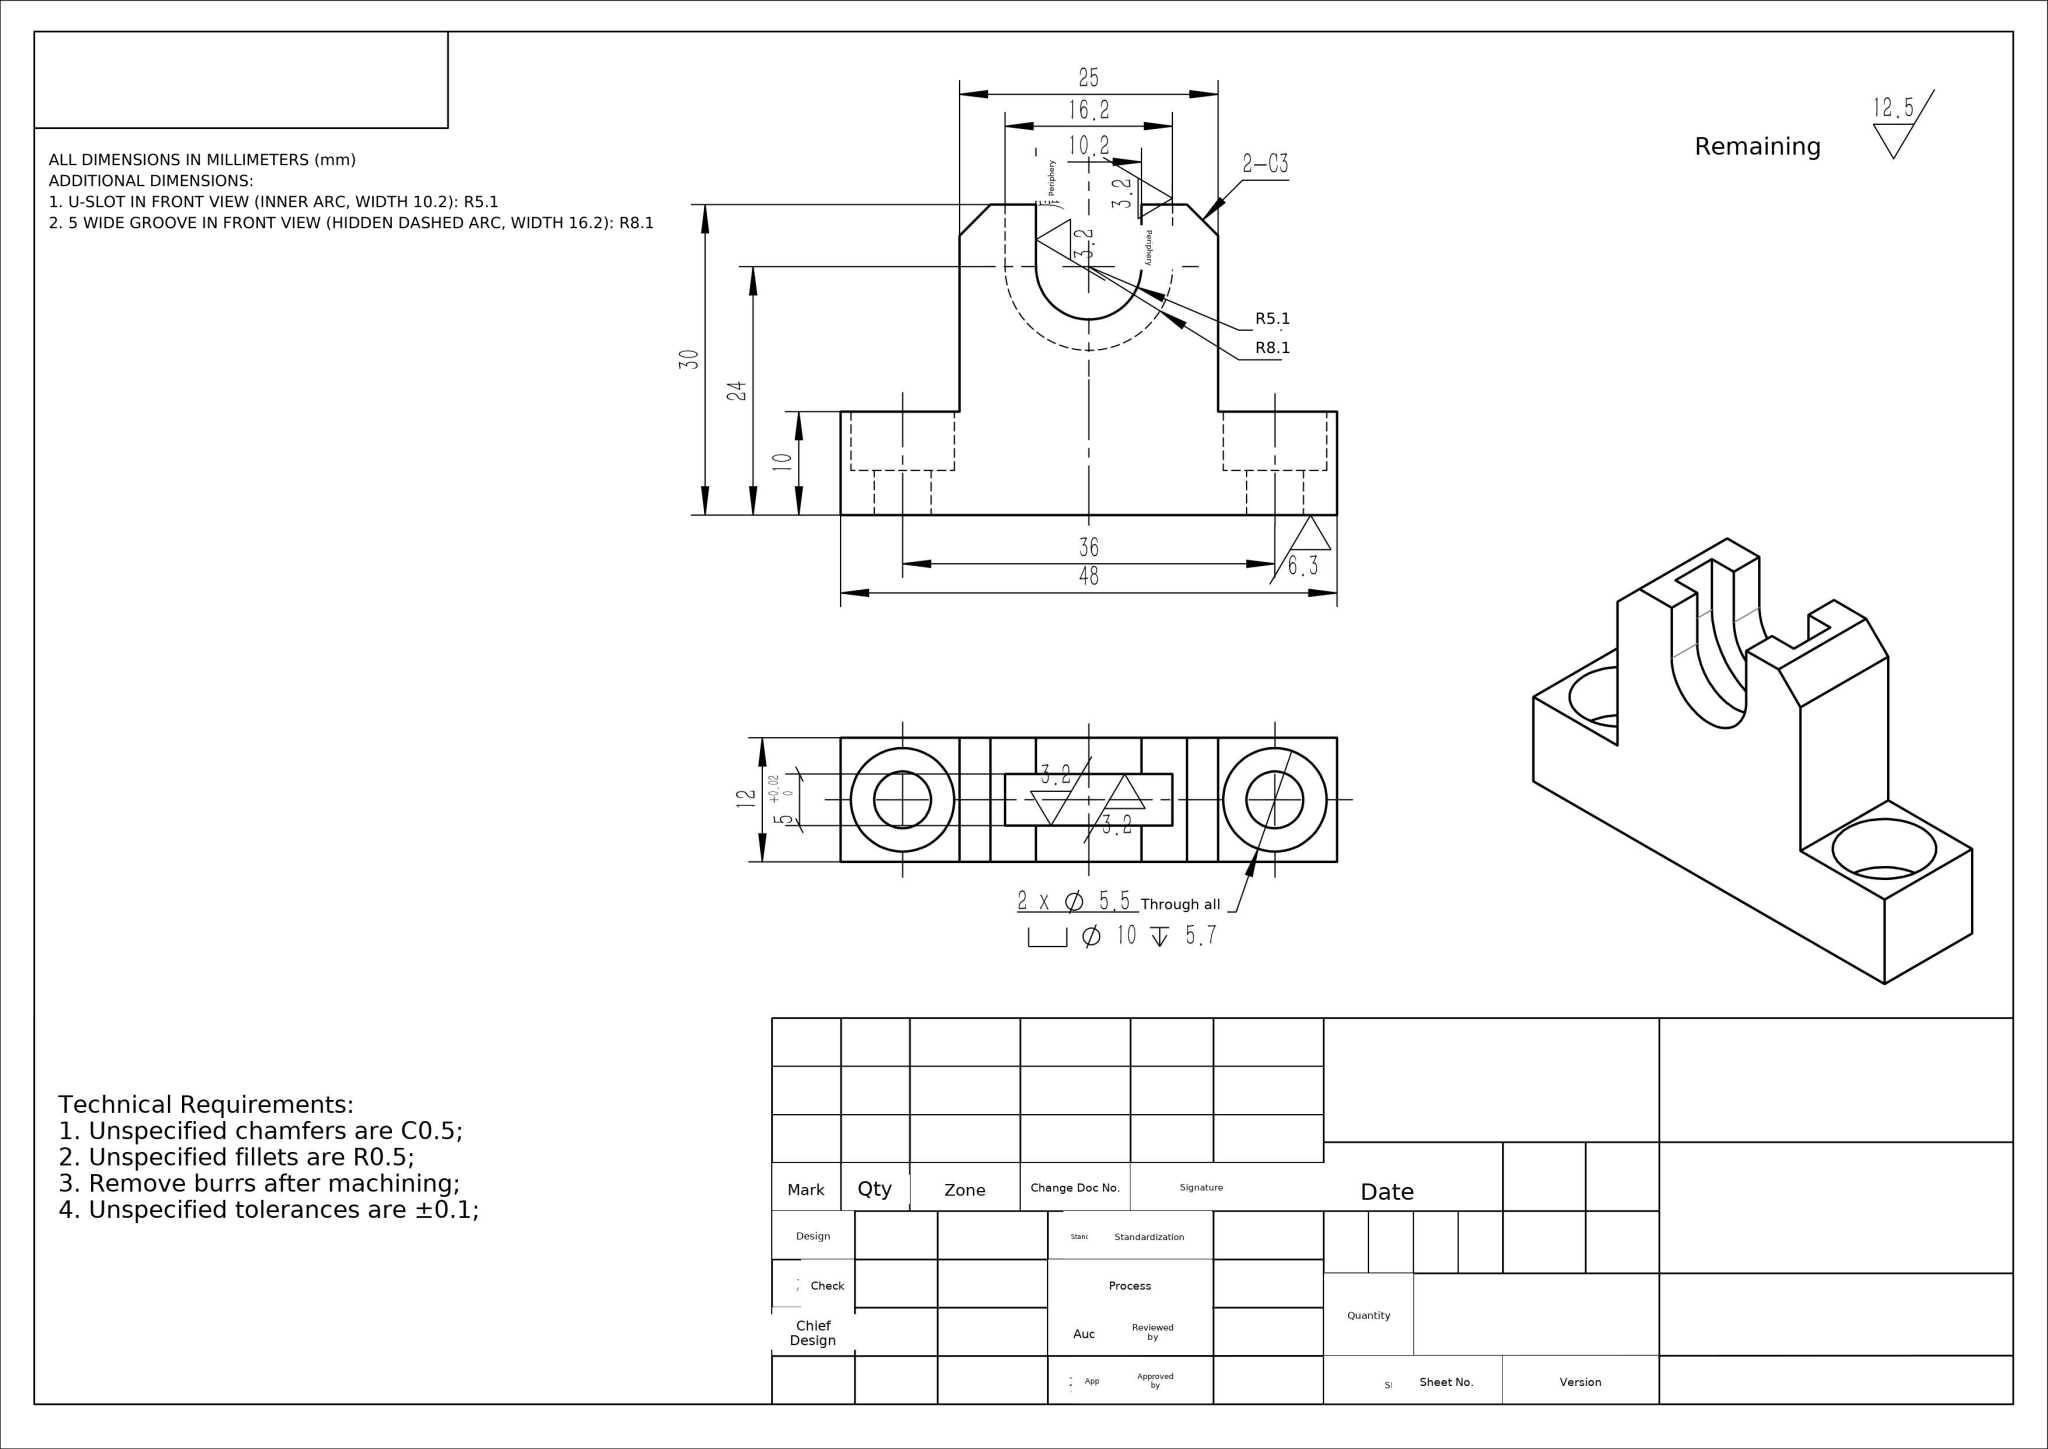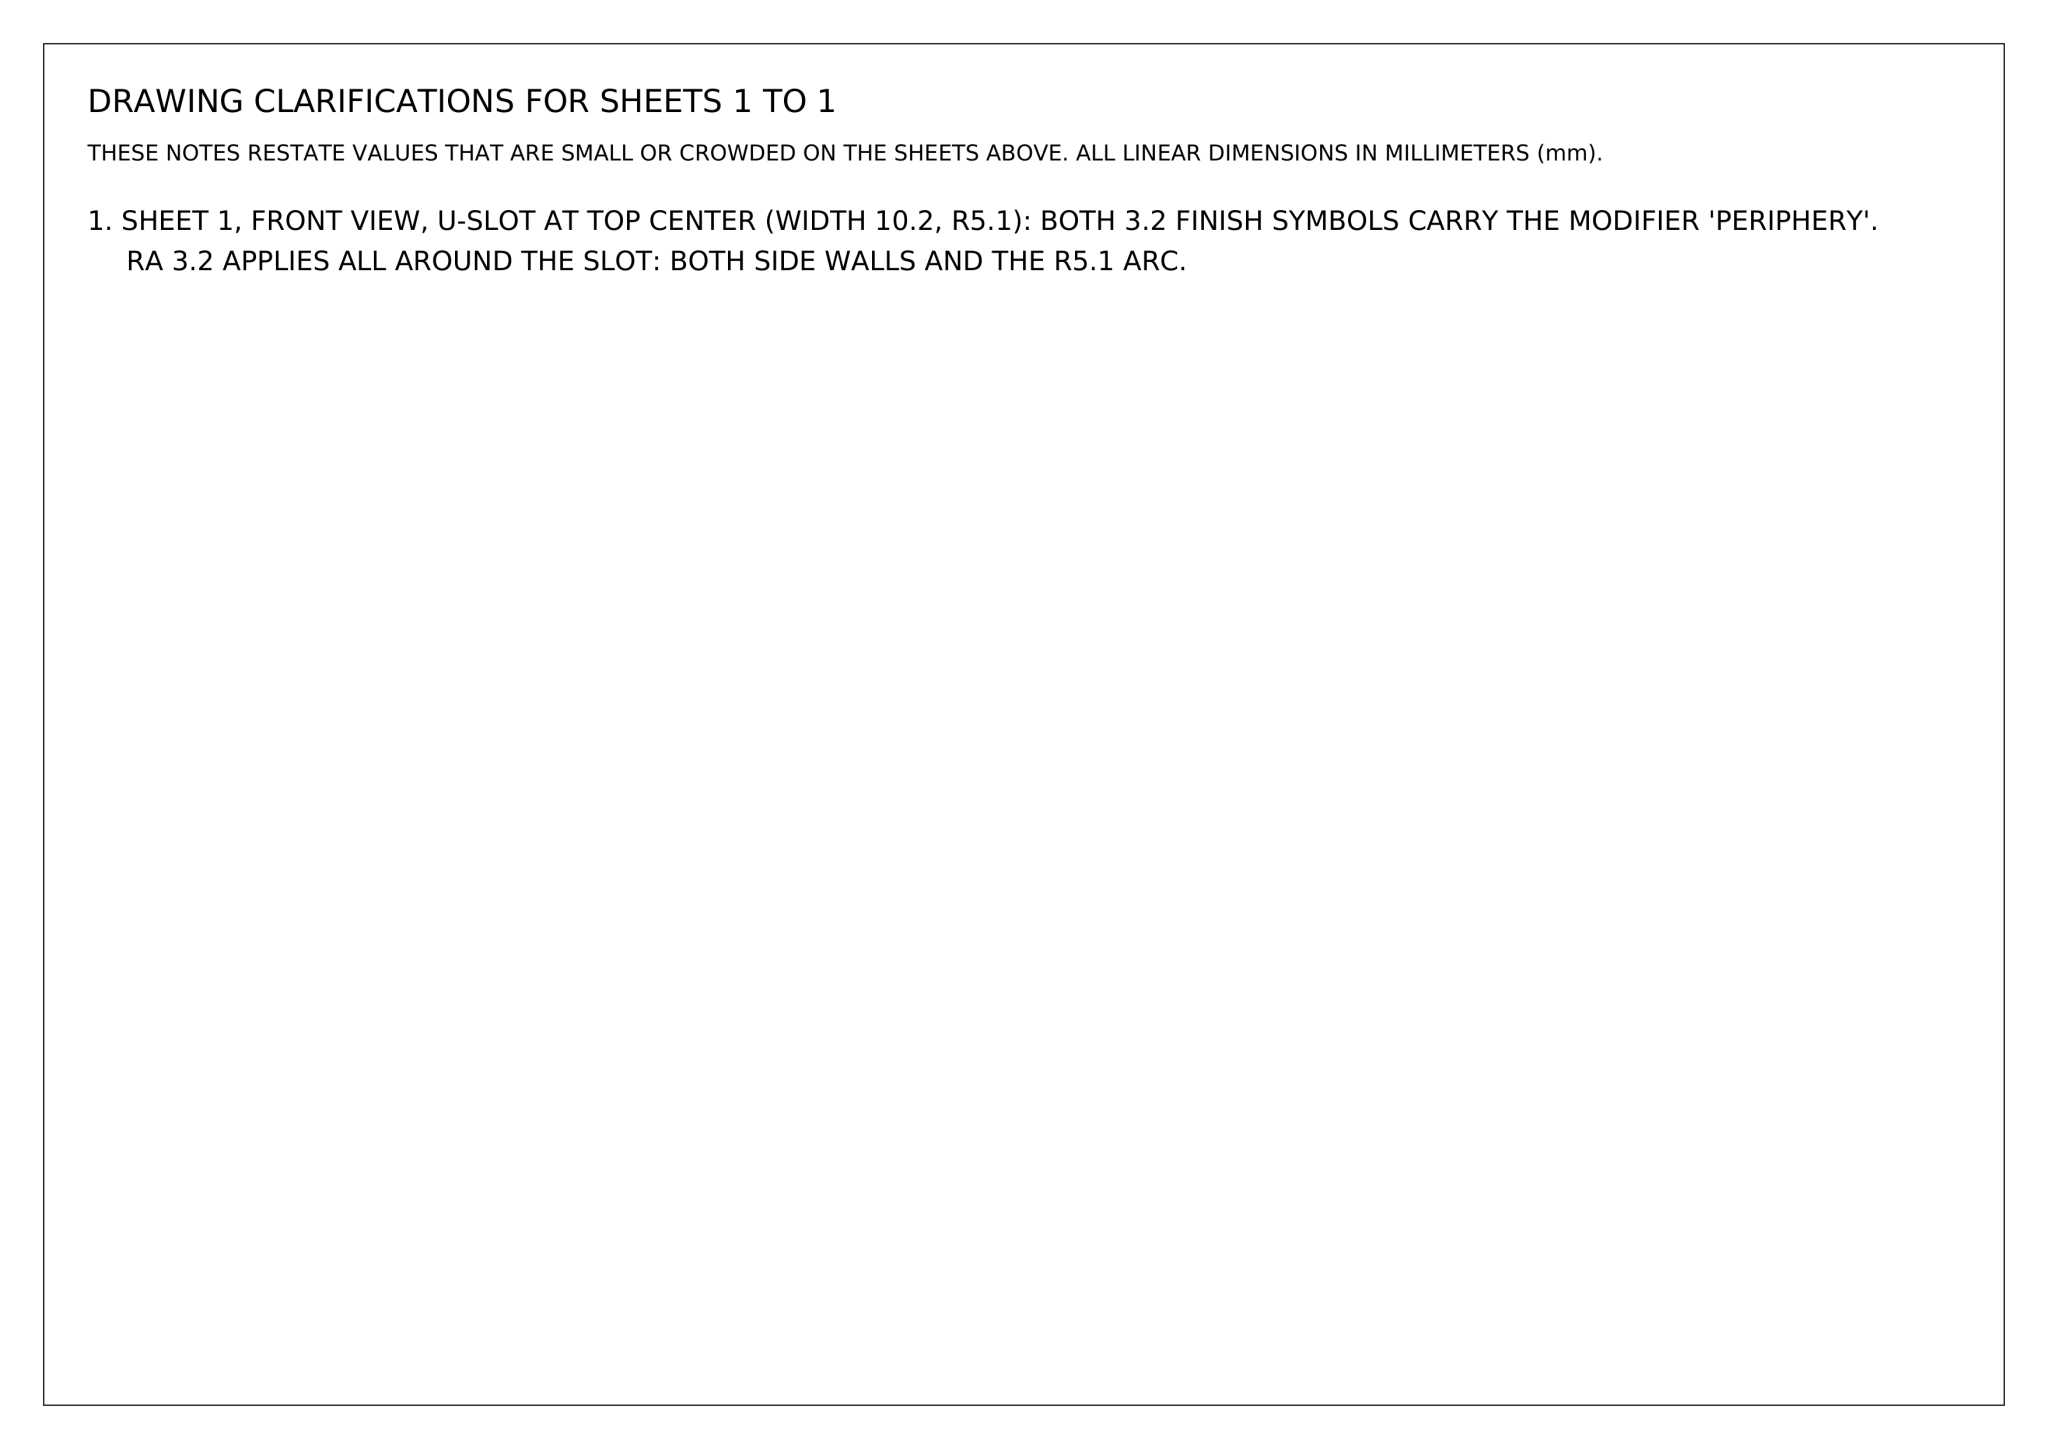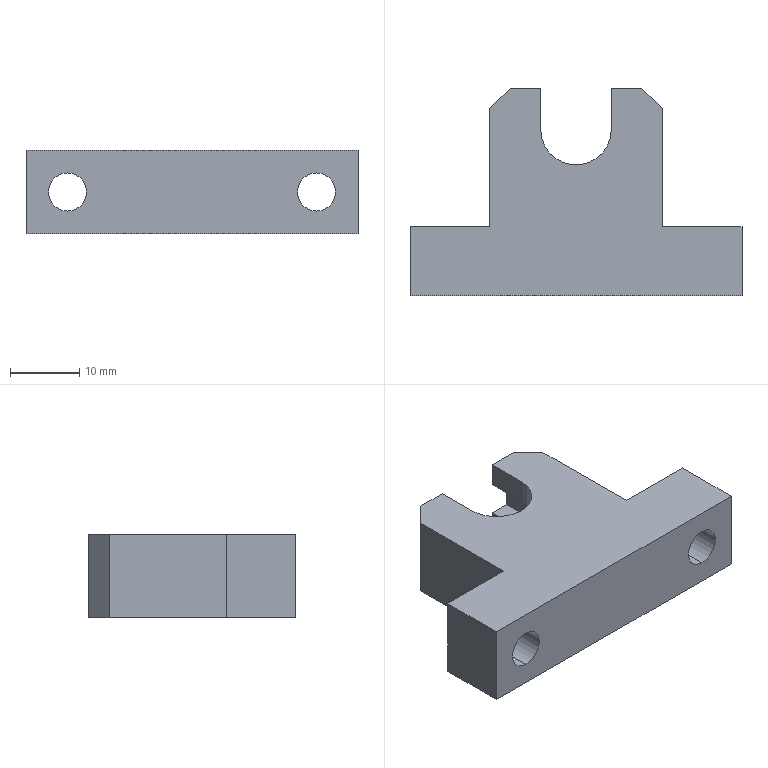Part | NX | mm | 1 solid | 34 faces | box 48 x 30 x 12 mm | volume 8837 mm3 | plane 23 | cylinder 11 | commonest cylinder face diameters 10 x4 5.5 x4 10.2 x2 16.2 x1